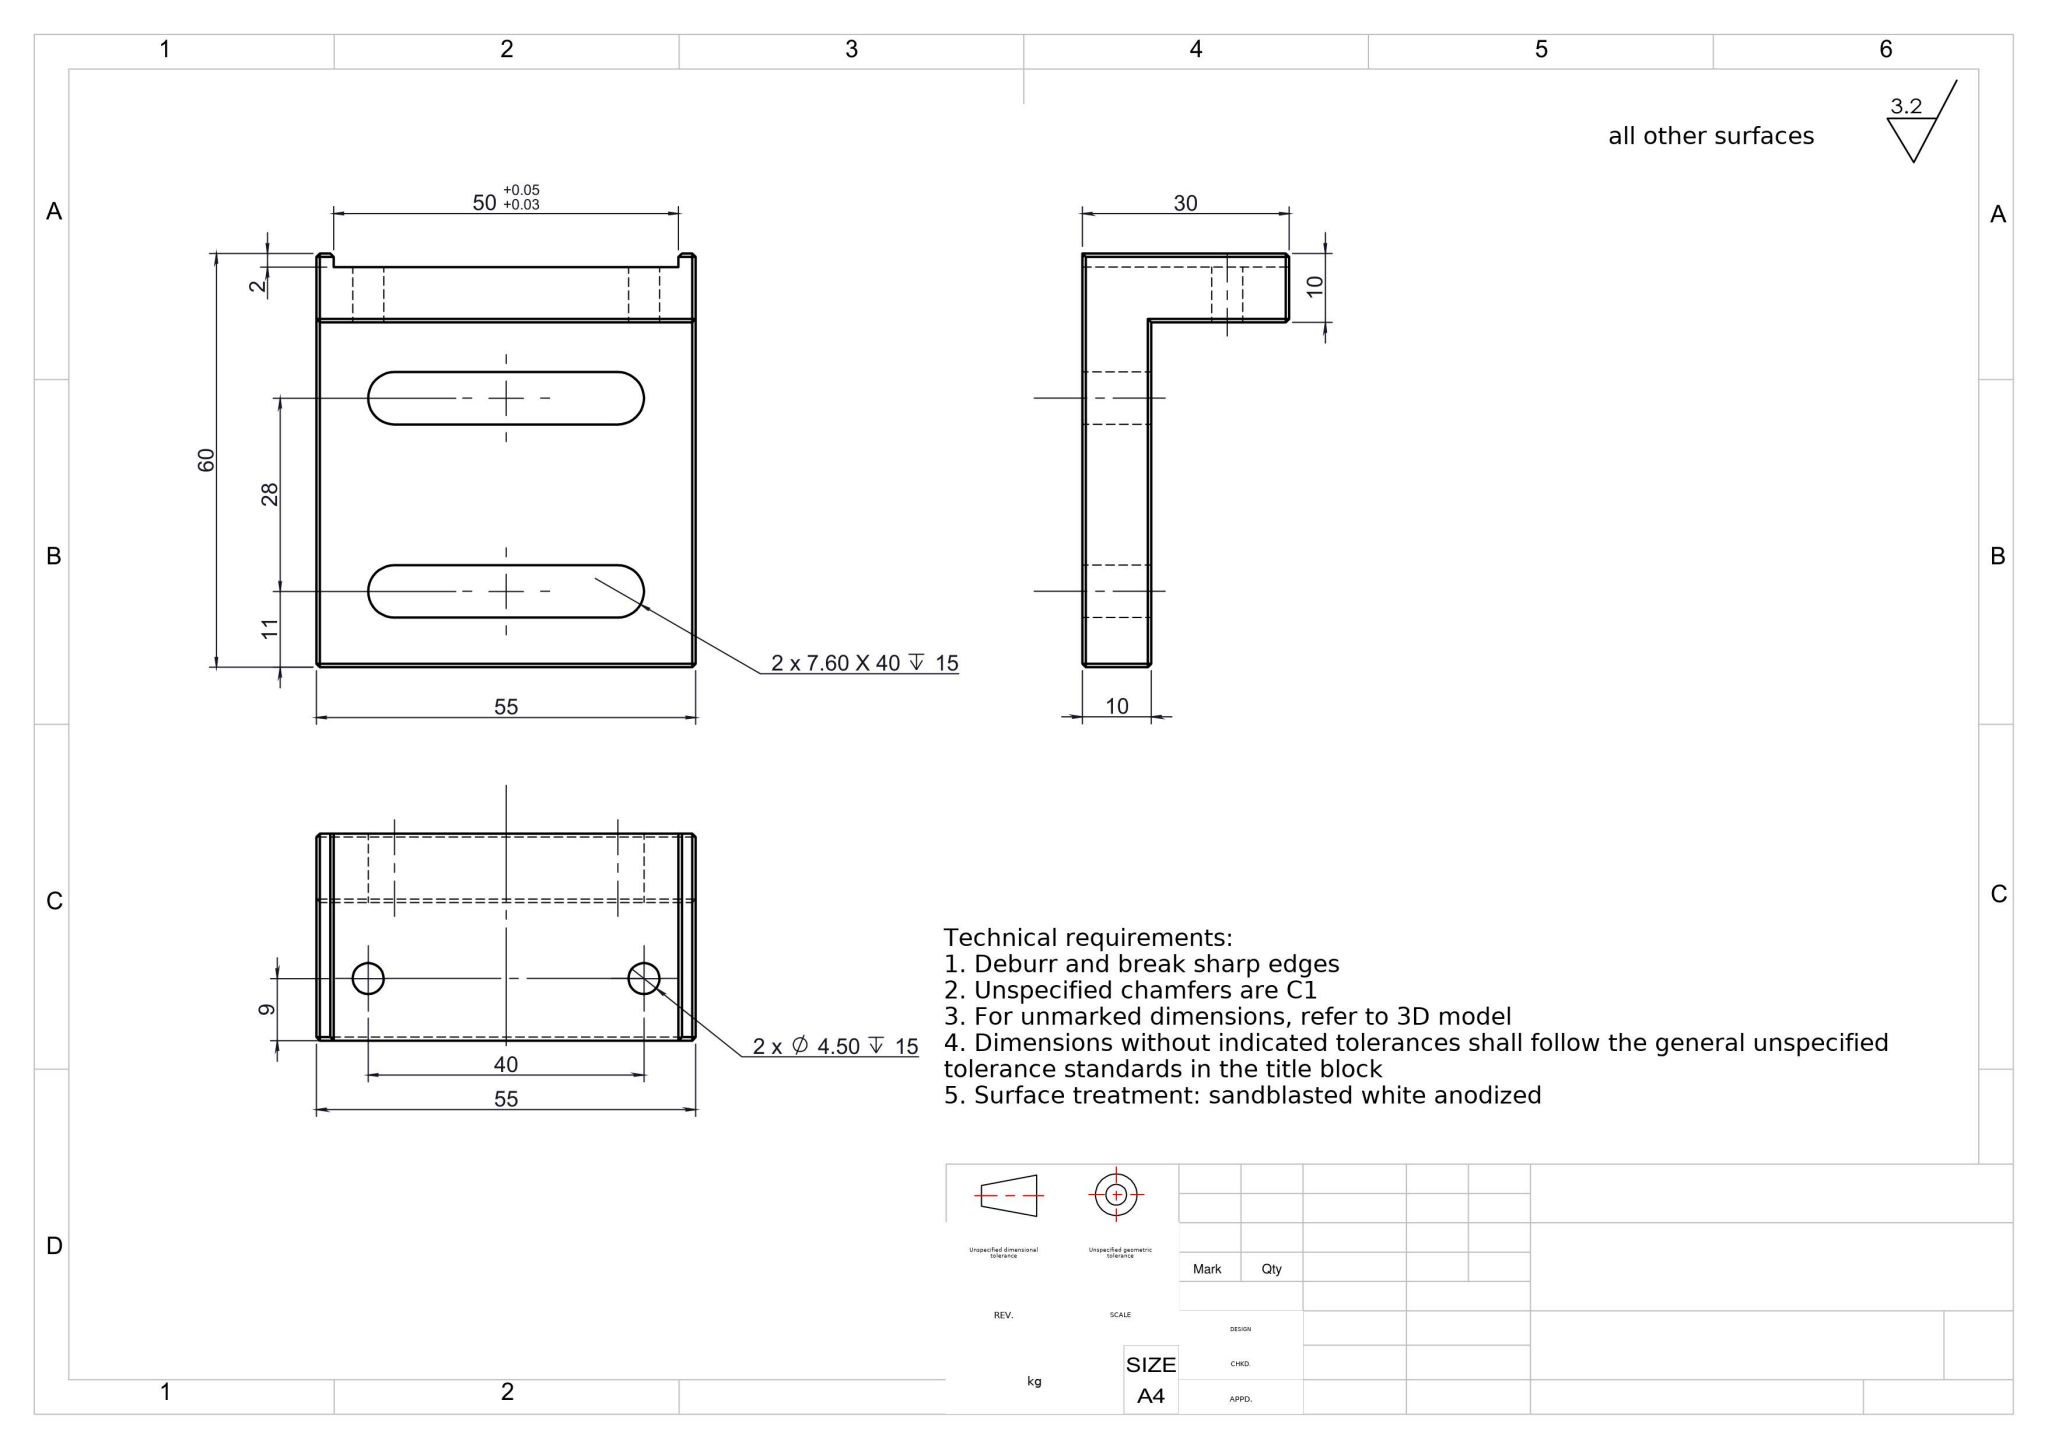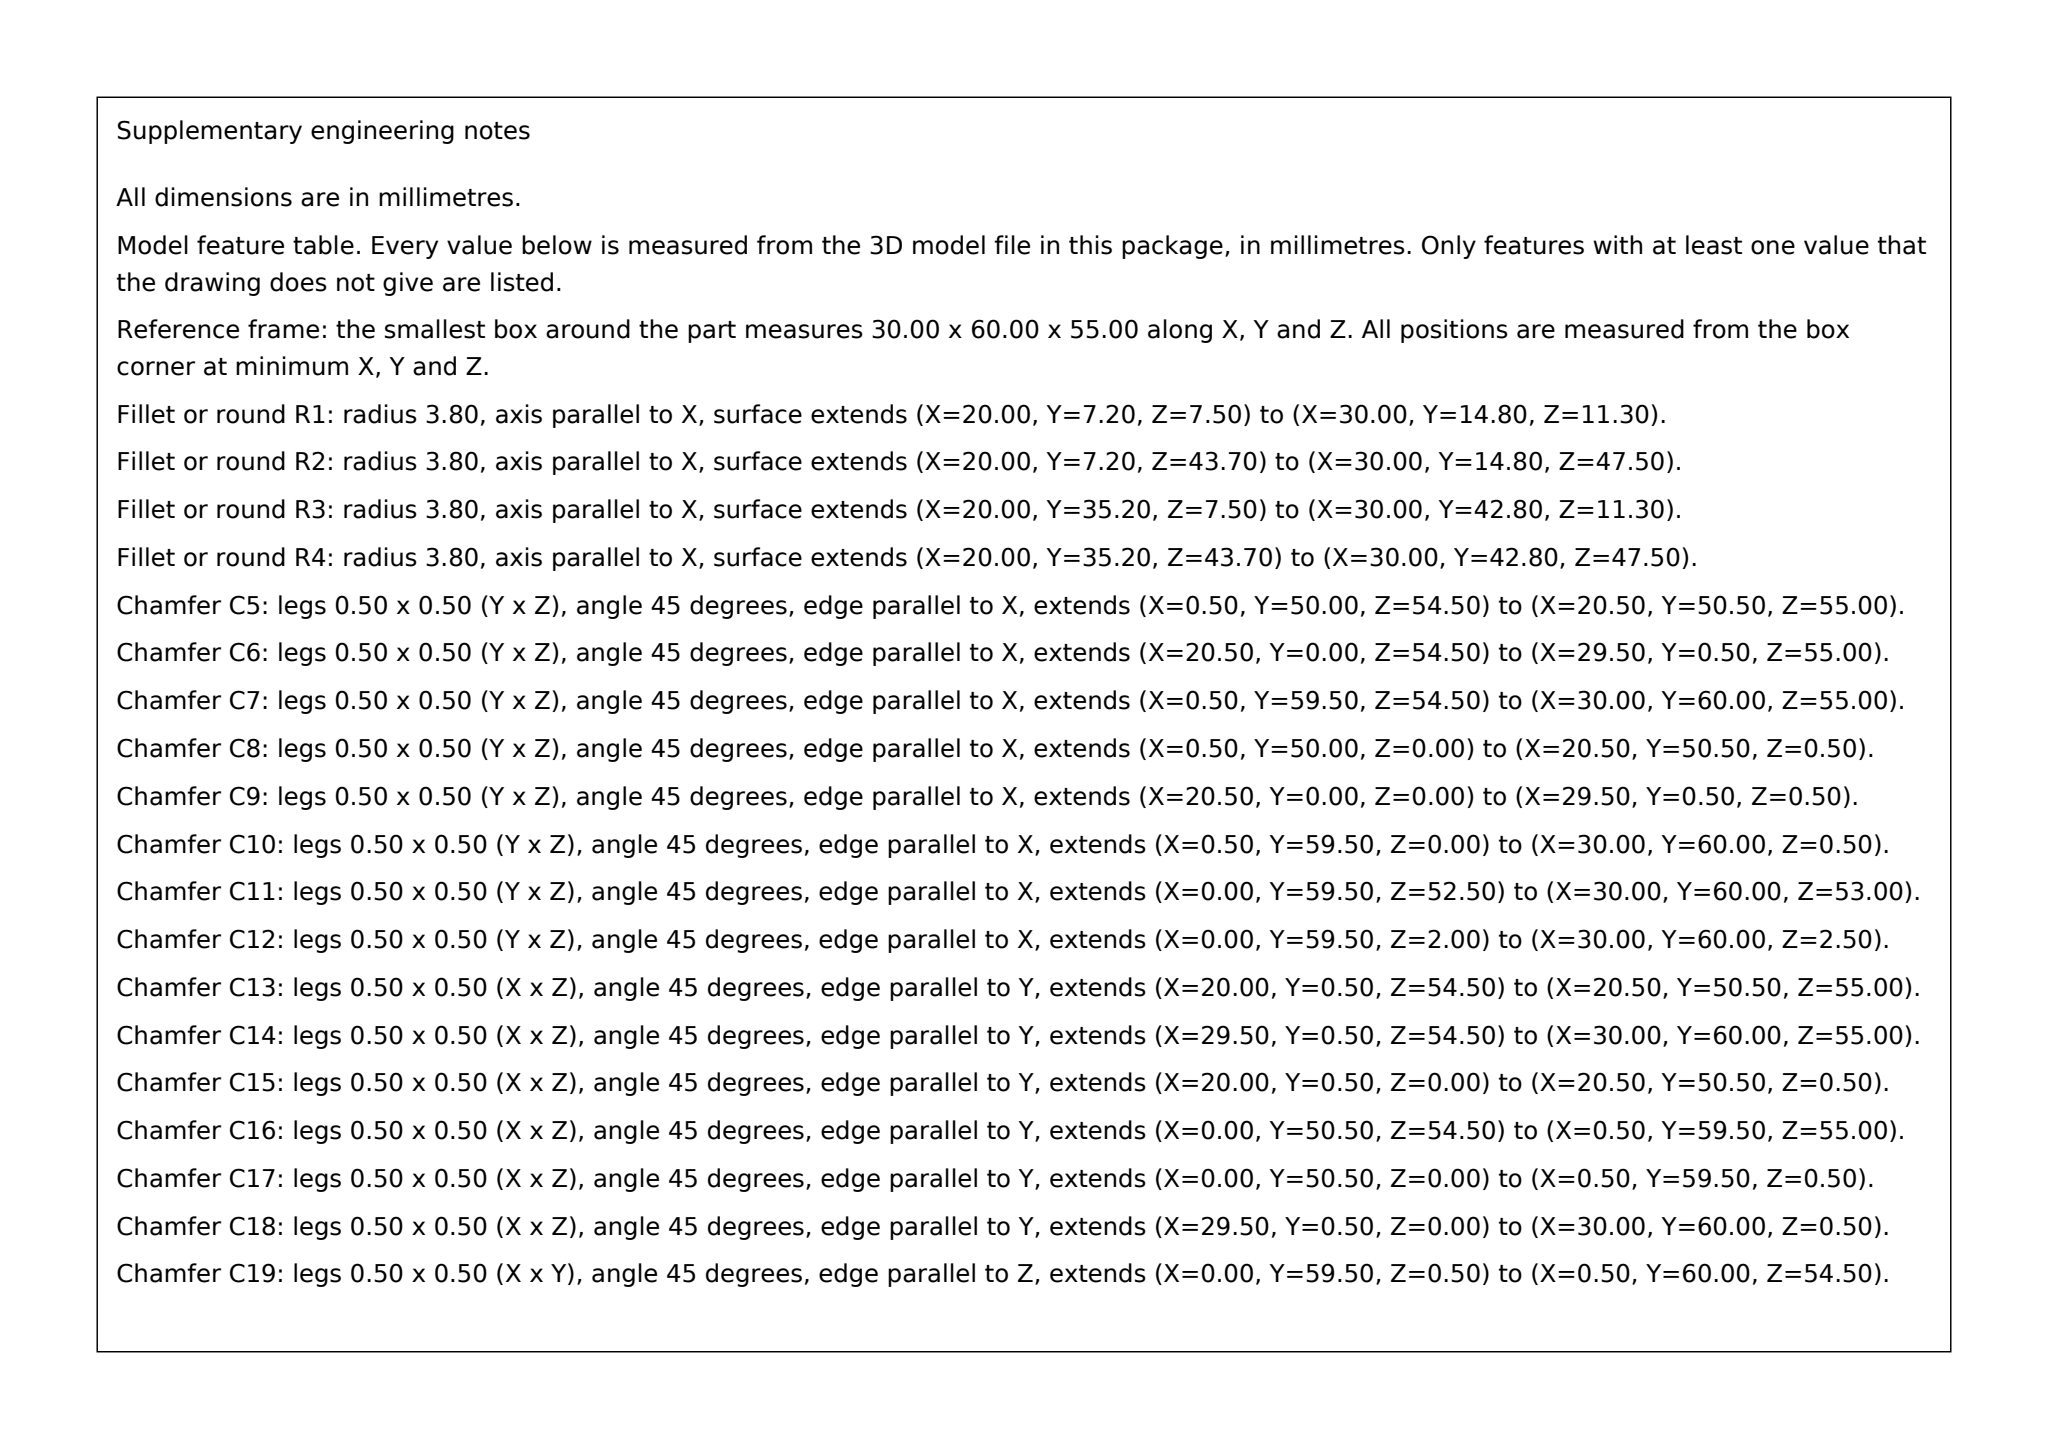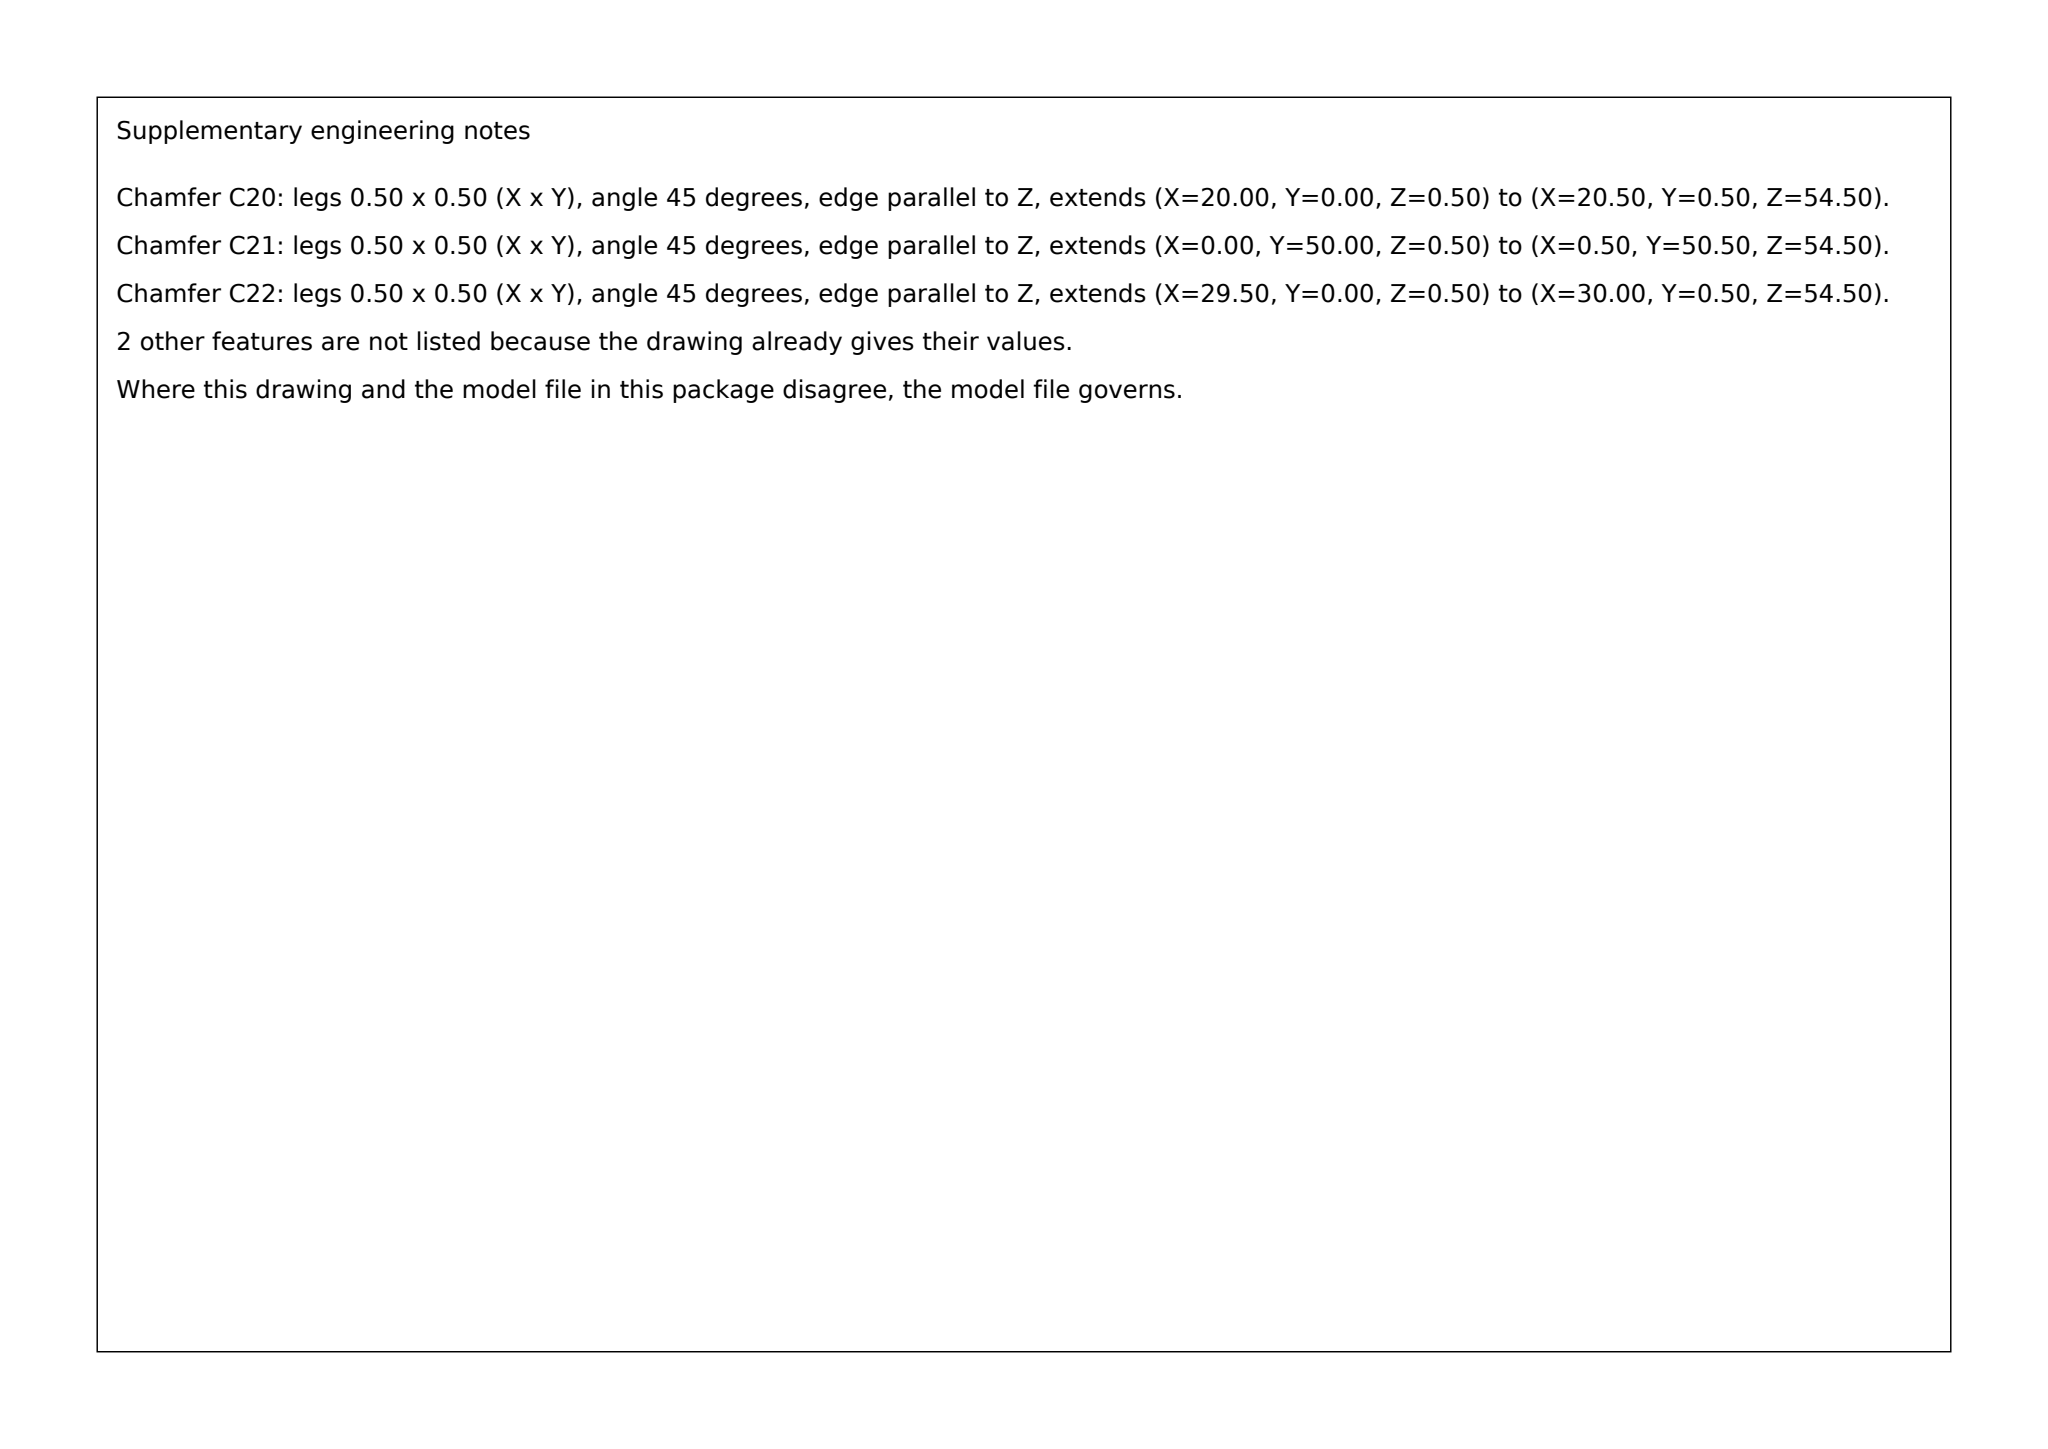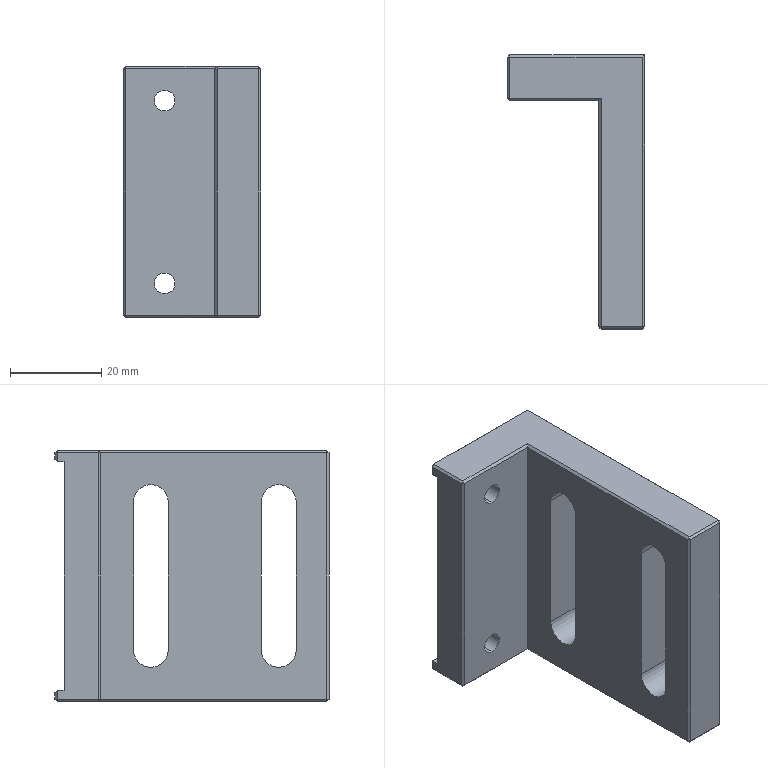Part | SolidWorks | mm | 1 solid | 53 faces | box 30 x 60 x 55 mm | volume 34840 mm3 | plane 43 | cylinder 10 | commonest cylinder face diameters 7.6 x6 4.5 x4